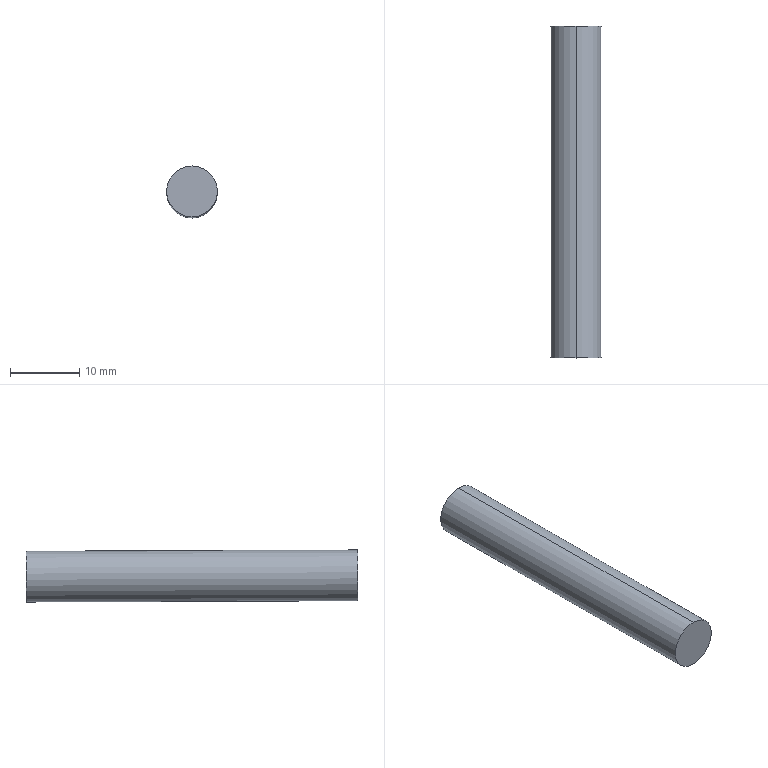Component | SolidWorks | RehabilitationChair-18-7-2 | 1 solid | 4 faces | box 7.34 x 47.96 x 7.52 mm | volume 2029 mm3 | cylinder 2 | plane 2 | commonest cylinder face diameters 7.342 x2
STEP:
#1=CARTESIAN_POINT('',(19.723,8.346,11.906));
#2=VERTEX_POINT('',#1);
#3=CARTESIAN_POINT('',(19.723,8.345,11.617));
#4=VERTEX_POINT('',#3);
#5=CARTESIAN_POINT('',(19.723,8.345,11.761));
#6=DIRECTION('',(-0.,1.,-0.003798));
#7=DIRECTION('',(0.,0.003798,1.));
#8=AXIS2_PLACEMENT_3D('',#5,#6,#7);
#9=CIRCLE('',#8,0.1445);
#10=EDGE_CURVE('',#2,#4,#9,.T.);
#11=ORIENTED_EDGE('',*,*,#10,.F.);
#12=CARTESIAN_POINT('',(19.723,6.459,11.913));
#13=VERTEX_POINT('',#12);
#14=CARTESIAN_POINT('',(19.723,8.388,11.906));
#15=DIRECTION('',(-0.,-1.,0.003798));
#16=VECTOR('',#15,39.37);
#17=LINE('',#14,#16);
#18=EDGE_CURVE('',#2,#13,#17,.T.);
#19=ORIENTED_EDGE('',*,*,#18,.T.);
#20=CARTESIAN_POINT('',(19.723,6.458,11.624));
#21=VERTEX_POINT('',#20);
#22=CARTESIAN_POINT('',(19.723,6.458,11.768));
#23=DIRECTION('',(0.,1.,-0.003798));
#24=DIRECTION('',(0.,0.003798,1.));
#25=AXIS2_PLACEMENT_3D('',#22,#23,#24);
#26=CIRCLE('',#25,0.1445);
#27=EDGE_CURVE('',#13,#21,#26,.T.);
#28=ORIENTED_EDGE('',*,*,#27,.T.);
#29=CARTESIAN_POINT('',(19.723,8.387,11.617));
#30=DIRECTION('',(-0.,-1.,0.003798));
#31=VECTOR('',#30,39.37);
#32=LINE('',#29,#31);
#33=EDGE_CURVE('',#4,#21,#32,.T.);
#34=ORIENTED_EDGE('',*,*,#33,.F.);
#35=EDGE_LOOP('',(#11,#19,#28,#34));
#36=FACE_OUTER_BOUND('',#35,.T.);
#37=CARTESIAN_POINT('',(19.723,8.387,11.761));
#38=DIRECTION('',(-0.,-1.,0.003798));
#39=DIRECTION('',(0.,-0.003798,-1.));
#40=AXIS2_PLACEMENT_3D('',#37,#38,#39);
#41=CYLINDRICAL_SURFACE('',#40,0.1445);
#42=ADVANCED_FACE('',(#36),#41,.T.);
#43=ORIENTED_EDGE('',*,*,#18,.F.);
#44=CARTESIAN_POINT('',(19.723,8.345,11.761));
#45=DIRECTION('',(-0.,1.,-0.003798));
#46=DIRECTION('',(0.,0.003798,1.));
#47=AXIS2_PLACEMENT_3D('',#44,#45,#46);
#48=CIRCLE('',#47,0.1445);
#49=EDGE_CURVE('',#4,#2,#48,.T.);
#50=ORIENTED_EDGE('',*,*,#49,.F.);
#51=ORIENTED_EDGE('',*,*,#33,.T.);
#52=CARTESIAN_POINT('',(19.723,6.458,11.768));
#53=DIRECTION('',(0.,1.,-0.003798));
#54=DIRECTION('',(0.,0.003798,1.));
#55=AXIS2_PLACEMENT_3D('',#52,#53,#54);
#56=CIRCLE('',#55,0.1445);
#57=EDGE_CURVE('',#21,#13,#56,.T.);
#58=ORIENTED_EDGE('',*,*,#57,.T.);
#59=EDGE_LOOP('',(#43,#50,#51,#58));
#60=FACE_OUTER_BOUND('',#59,.T.);
#61=CARTESIAN_POINT('',(19.723,8.387,11.761));
#62=DIRECTION('',(-0.,-1.,0.003798));
#63=DIRECTION('',(0.,-0.003798,-1.));
#64=AXIS2_PLACEMENT_3D('',#61,#62,#63);
#65=CYLINDRICAL_SURFACE('',#64,0.1445);
#66=ADVANCED_FACE('',(#60),#65,.T.);
#67=ORIENTED_EDGE('',*,*,#57,.F.);
#68=ORIENTED_EDGE('',*,*,#27,.F.);
#69=EDGE_LOOP('',(#67,#68));
#70=FACE_OUTER_BOUND('',#69,.T.);
#71=CARTESIAN_POINT('',(19.723,6.458,11.768));
#72=DIRECTION('',(0.,1.,-0.003798));
#73=DIRECTION('',(-0.,0.003798,1.));
#74=AXIS2_PLACEMENT_3D('',#71,#72,#73);
#75=PLANE('',#74);
#76=ADVANCED_FACE('',(#70),#75,.F.);
#77=ORIENTED_EDGE('',*,*,#49,.T.);
#78=ORIENTED_EDGE('',*,*,#10,.T.);
#79=EDGE_LOOP('',(#77,#78));
#80=FACE_OUTER_BOUND('',#79,.T.);
#81=CARTESIAN_POINT('',(-0.,8.39,23.554));
#82=DIRECTION('',(-0.,1.,-0.003798));
#83=DIRECTION('',(-0.,0.003798,1.));
#84=AXIS2_PLACEMENT_3D('',#81,#82,#83);
#85=PLANE('',#84);
#86=ADVANCED_FACE('',(#80),#85,.T.);
#87=CLOSED_SHELL('',(#42,#66,#76,#86));
#88=MANIFOLD_SOLID_BREP('',#87);
#89=CARTESIAN_POINT('',(0.,0.,0.));
#90=DIRECTION('',(0.,0.,1.));
#91=DIRECTION('',(1.,0.,0.));
#92=AXIS2_PLACEMENT_3D('',#89,#90,#91);
#93=(LENGTH_UNIT()NAMED_UNIT(*)SI_UNIT($,.METRE.));
#94=LENGTH_MEASURE_WITH_UNIT(LENGTH_MEASURE(0.0254),#93);
#95=DIMENSIONAL_EXPONENTS(1.,0.,0.,0.,0.,0.,0.);
#96=(CONVERSION_BASED_UNIT('',#94)LENGTH_UNIT()NAMED_UNIT(#95));
#97=UNCERTAINTY_MEASURE_WITH_UNIT(LENGTH_MEASURE(0.00001),#96,'','');
#98=(NAMED_UNIT(*)PLANE_ANGLE_UNIT()SI_UNIT($,.RADIAN.));
#99=(NAMED_UNIT(*)SI_UNIT($,.STERADIAN.)SOLID_ANGLE_UNIT());
#100=(GEOMETRIC_REPRESENTATION_CONTEXT(3)GLOBAL_UNCERTAINTY_ASSIGNED_CONTEXT((#97))GLOBAL_UNIT_ASSIGNED_CONTEXT((#96,#98,#99))REPRESENTATION_CONTEXT('',''));
#101=ADVANCED_BREP_SHAPE_REPRESENTATION('',(#88,#92),#100);
#102=COLOUR_RGB('',0.7922,0.8196,0.9333);
#103=FILL_AREA_STYLE_COLOUR('',#102);
#104=FILL_AREA_STYLE('',(#103));
#105=SURFACE_STYLE_FILL_AREA(#104);
#106=SURFACE_SIDE_STYLE('',(#105));
#107=SURFACE_STYLE_USAGE(.BOTH.,#106);
#108=PRESENTATION_STYLE_ASSIGNMENT((#107));
#109=STYLED_ITEM('',(#108),#88);
#110=PRESENTATION_LAYER_ASSIGNMENT('','',(#109));
#111=(LENGTH_UNIT()NAMED_UNIT(*)SI_UNIT($,.METRE.));
#112=LENGTH_MEASURE_WITH_UNIT(LENGTH_MEASURE(0.0254),#111);
#113=DIMENSIONAL_EXPONENTS(1.,0.,0.,0.,0.,0.,0.);
#114=(CONVERSION_BASED_UNIT('',#112)LENGTH_UNIT()NAMED_UNIT(#113));
#115=UNCERTAINTY_MEASURE_WITH_UNIT(LENGTH_MEASURE(0.00001),#114,'','');
#116=(NAMED_UNIT(*)PLANE_ANGLE_UNIT()SI_UNIT($,.RADIAN.));
#117=(NAMED_UNIT(*)SI_UNIT($,.STERADIAN.)SOLID_ANGLE_UNIT());
#118=(GEOMETRIC_REPRESENTATION_CONTEXT(3)GLOBAL_UNCERTAINTY_ASSIGNED_CONTEXT((#115))GLOBAL_UNIT_ASSIGNED_CONTEXT((#114,#116,#117))REPRESENTATION_CONTEXT('',''));
#119=MECHANICAL_DESIGN_GEOMETRIC_PRESENTATION_REPRESENTATION('',(#109),#118);